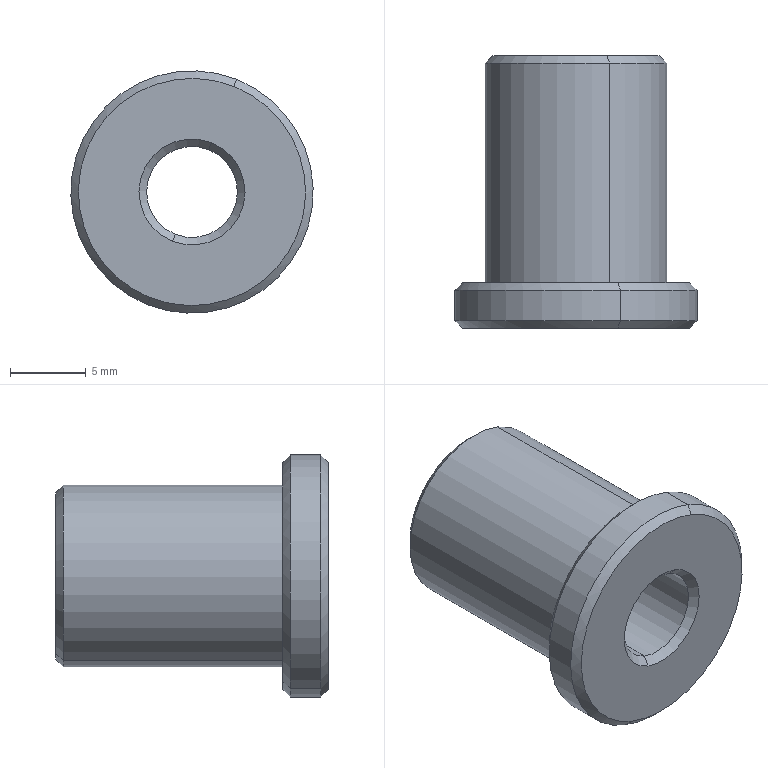Component | SolidWorks | GbgbSleeve-1 | 1 solid | 19 faces | box 16 x 18 x 16 mm | volume 1769 mm3 | cone 10 | cylinder 6 | plane 3 | commonest cylinder face diameters 6 x2 12 x2 16 x2
build123d program:
from build123d import *

# Parameters (mm, degrees)
SKETCH1_R           = 8
BOSS_EXTRUDE1_DEPTH = 3
SKETCH2_R           = 6
BOSS_EXTRUDE2_DEPTH = 15
SKETCH3_R           = 3
CUT_EXTRUDE1_DEPTH  = 22.26
CHAMFER1_SIZE       = 0.5


with BuildPart() as part:
    # Sketch1 → Boss-Extrude1 (new body)
    with BuildSketch(Plane(origin=(0, 0, 0), x_dir=(1, 0, 0), z_dir=(0, 1, 0))):
        with Locations(Location((0, 0, 0), (0, 0, 270))):
            Circle(SKETCH1_R)
    extrude(amount=BOSS_EXTRUDE1_DEPTH)

    # Sketch2 → Boss-Extrude2 (add)
    with BuildSketch(Plane(origin=(0, 3, 0), x_dir=(1, 0, 0), z_dir=(0, 1, 0))):
        with Locations(Location((0, 0, 0), (0, 0, 270))):
            Circle(SKETCH2_R)
    extrude(amount=BOSS_EXTRUDE2_DEPTH)

    # Sketch3 → Cut-Extrude1 (cut, through all)
    with BuildSketch(Plane(origin=(0, 18, 0), x_dir=(1, 0, 0), z_dir=(0, 1, 0))):
        with Locations(Location((0, 0, 0), (0, 0, 270))):
            Circle(SKETCH3_R)
    extrude(amount=-CUT_EXTRUDE1_DEPTH, mode=Mode.SUBTRACT)

    # Chamfer1
    chamfer1_edges = [part.edges().sort_by_distance(p)[0] for p in [
        (0, 0, -3),
        (0, 18, -3),
        (0, 0, -8),
        (0, 3, -8),
        (0, 18, -6),
    ]]
    chamfer(chamfer1_edges, length=CHAMFER1_SIZE)


solid = part.part

# Placed as in the assembly
solid = solid.moved(Location((55.446, 369.44, 430.232), (0, 0, 0)))
STEP:
#1=COLOUR_RGB('',0.7922,0.8196,0.9333);
#2=FILL_AREA_STYLE_COLOUR('',#1);
#3=FILL_AREA_STYLE('',(#2));
#4=SURFACE_STYLE_FILL_AREA(#3);
#5=SURFACE_SIDE_STYLE('',(#4));
#6=SURFACE_STYLE_USAGE(.BOTH.,#5);
#7=PRESENTATION_STYLE_ASSIGNMENT((#6));
#8=CARTESIAN_POINT('',(2.263,15.254,17.14));
#9=VERTEX_POINT('',#8);
#10=CARTESIAN_POINT('',(2.103,15.254,16.737));
#11=VERTEX_POINT('',#10);
#12=CARTESIAN_POINT('',(2.183,15.254,16.938));
#13=DIRECTION('',(-0.,1.,0.));
#14=DIRECTION('',(0.3675,0.,0.93));
#15=AXIS2_PLACEMENT_3D('',#12,#13,#14);
#16=CIRCLE('',#15,0.2165);
#17=EDGE_CURVE('',#9,#11,#16,.T.);
#18=ORIENTED_EDGE('',*,*,#17,.F.);
#19=CARTESIAN_POINT('',(2.27,15.234,17.158));
#20=VERTEX_POINT('',#19);
#21=CARTESIAN_POINT('',(2.263,15.254,17.14));
#22=DIRECTION('',(0.2599,-0.7071,0.6576));
#23=VECTOR('',#22,39.37);
#24=LINE('',#21,#23);
#25=EDGE_CURVE('',#9,#20,#24,.T.);
#26=ORIENTED_EDGE('',*,*,#25,.T.);
#27=CARTESIAN_POINT('',(2.096,15.234,16.719));
#28=VERTEX_POINT('',#27);
#29=CARTESIAN_POINT('',(2.183,15.234,16.938));
#30=DIRECTION('',(0.,-1.,-0.));
#31=DIRECTION('',(0.3675,0.,0.93));
#32=AXIS2_PLACEMENT_3D('',#29,#30,#31);
#33=CIRCLE('',#32,0.2362);
#34=EDGE_CURVE('',#28,#20,#33,.T.);
#35=ORIENTED_EDGE('',*,*,#34,.F.);
#36=CARTESIAN_POINT('',(2.103,15.254,16.737));
#37=DIRECTION('',(-0.2599,-0.7071,-0.6576));
#38=VECTOR('',#37,39.37);
#39=LINE('',#36,#38);
#40=EDGE_CURVE('',#11,#28,#39,.T.);
#41=ORIENTED_EDGE('',*,*,#40,.F.);
#42=EDGE_LOOP('',(#18,#26,#35,#41));
#43=FACE_OUTER_BOUND('',#42,.T.);
#44=CARTESIAN_POINT('',(2.183,15.254,16.938));
#45=DIRECTION('',(0.,-1.,-0.));
#46=DIRECTION('',(-0.3675,0.,-0.93));
#47=AXIS2_PLACEMENT_3D('',#44,#45,#46);
#48=CONICAL_SURFACE('',#47,0.2165,0.7854);
#49=ADVANCED_FACE('',(#43),#48,.T.);
#50=CARTESIAN_POINT('',(2.291,14.663,17.213));
#51=VERTEX_POINT('',#50);
#52=CARTESIAN_POINT('',(2.074,14.663,16.664));
#53=VERTEX_POINT('',#52);
#54=CARTESIAN_POINT('',(2.183,14.663,16.938));
#55=DIRECTION('',(-0.,1.,0.));
#56=DIRECTION('',(0.3675,0.,0.93));
#57=AXIS2_PLACEMENT_3D('',#54,#55,#56);
#58=CIRCLE('',#57,0.2953);
#59=EDGE_CURVE('',#51,#53,#58,.T.);
#60=ORIENTED_EDGE('',*,*,#59,.F.);
#61=CARTESIAN_POINT('',(2.299,14.643,17.231));
#62=VERTEX_POINT('',#61);
#63=CARTESIAN_POINT('',(2.291,14.663,17.213));
#64=DIRECTION('',(0.2599,-0.7071,0.6576));
#65=VECTOR('',#64,39.37);
#66=LINE('',#63,#65);
#67=EDGE_CURVE('',#51,#62,#66,.T.);
#68=ORIENTED_EDGE('',*,*,#67,.T.);
#69=CARTESIAN_POINT('',(2.067,14.643,16.645));
#70=VERTEX_POINT('',#69);
#71=CARTESIAN_POINT('',(2.183,14.643,16.938));
#72=DIRECTION('',(0.,-1.,-0.));
#73=DIRECTION('',(0.3675,0.,0.93));
#74=AXIS2_PLACEMENT_3D('',#71,#72,#73);
#75=CIRCLE('',#74,0.315);
#76=EDGE_CURVE('',#70,#62,#75,.T.);
#77=ORIENTED_EDGE('',*,*,#76,.F.);
#78=CARTESIAN_POINT('',(2.074,14.663,16.664));
#79=DIRECTION('',(-0.2599,-0.7071,-0.6576));
#80=VECTOR('',#79,39.37);
#81=LINE('',#78,#80);
#82=EDGE_CURVE('',#53,#70,#81,.T.);
#83=ORIENTED_EDGE('',*,*,#82,.F.);
#84=EDGE_LOOP('',(#60,#68,#77,#83));
#85=FACE_OUTER_BOUND('',#84,.T.);
#86=CARTESIAN_POINT('',(2.183,14.663,16.938));
#87=DIRECTION('',(0.,-1.,-0.));
#88=DIRECTION('',(-0.3675,0.,-0.93));
#89=AXIS2_PLACEMENT_3D('',#86,#87,#88);
#90=CONICAL_SURFACE('',#89,0.2953,0.7854);
#91=ADVANCED_FACE('',(#85),#90,.T.);
#92=CARTESIAN_POINT('',(2.074,14.545,16.664));
#93=VERTEX_POINT('',#92);
#94=CARTESIAN_POINT('',(2.291,14.545,17.213));
#95=VERTEX_POINT('',#94);
#96=CARTESIAN_POINT('',(2.183,14.545,16.938));
#97=DIRECTION('',(0.,-1.,-0.));
#98=DIRECTION('',(0.3675,0.,0.93));
#99=AXIS2_PLACEMENT_3D('',#96,#97,#98);
#100=CIRCLE('',#99,0.2953);
#101=EDGE_CURVE('',#93,#95,#100,.T.);
#102=ORIENTED_EDGE('',*,*,#101,.F.);
#103=CARTESIAN_POINT('',(2.067,14.565,16.645));
#104=VERTEX_POINT('',#103);
#105=CARTESIAN_POINT('',(2.067,14.565,16.645));
#106=DIRECTION('',(-0.2599,0.7071,-0.6576));
#107=VECTOR('',#106,39.37);
#108=LINE('',#105,#107);
#109=EDGE_CURVE('',#93,#104,#108,.T.);
#110=ORIENTED_EDGE('',*,*,#109,.T.);
#111=CARTESIAN_POINT('',(2.299,14.565,17.231));
#112=VERTEX_POINT('',#111);
#113=CARTESIAN_POINT('',(2.183,14.565,16.938));
#114=DIRECTION('',(-0.,1.,0.));
#115=DIRECTION('',(0.3675,0.,0.93));
#116=AXIS2_PLACEMENT_3D('',#113,#114,#115);
#117=CIRCLE('',#116,0.315);
#118=EDGE_CURVE('',#112,#104,#117,.T.);
#119=ORIENTED_EDGE('',*,*,#118,.F.);
#120=CARTESIAN_POINT('',(2.299,14.565,17.231));
#121=DIRECTION('',(0.2599,0.7071,0.6576));
#122=VECTOR('',#121,39.37);
#123=LINE('',#120,#122);
#124=EDGE_CURVE('',#95,#112,#123,.T.);
#125=ORIENTED_EDGE('',*,*,#124,.F.);
#126=EDGE_LOOP('',(#102,#110,#119,#125));
#127=FACE_OUTER_BOUND('',#126,.T.);
#128=CARTESIAN_POINT('',(2.183,14.565,16.938));
#129=DIRECTION('',(-0.,1.,0.));
#130=DIRECTION('',(0.3675,0.,0.93));
#131=AXIS2_PLACEMENT_3D('',#128,#129,#130);
#132=CONICAL_SURFACE('',#131,0.315,0.7854);
#133=ADVANCED_FACE('',(#127),#132,.T.);
#134=CARTESIAN_POINT('',(2.226,14.565,17.048));
#135=VERTEX_POINT('',#134);
#136=CARTESIAN_POINT('',(2.14,14.565,16.828));
#137=VERTEX_POINT('',#136);
#138=CARTESIAN_POINT('',(2.183,14.565,16.938));
#139=DIRECTION('',(0.,-1.,-0.));
#140=DIRECTION('',(0.3675,0.,0.93));
#141=AXIS2_PLACEMENT_3D('',#138,#139,#140);
#142=CIRCLE('',#141,0.1181);
#143=EDGE_CURVE('',#135,#137,#142,.T.);
#144=ORIENTED_EDGE('',*,*,#143,.F.);
#145=CARTESIAN_POINT('',(2.234,14.545,17.066));
#146=VERTEX_POINT('',#145);
#147=CARTESIAN_POINT('',(2.234,14.545,17.066));
#148=DIRECTION('',(0.2599,-0.7071,0.6576));
#149=VECTOR('',#148,39.37);
#150=LINE('',#147,#149);
#151=EDGE_CURVE('',#135,#146,#150,.T.);
#152=ORIENTED_EDGE('',*,*,#151,.T.);
#153=CARTESIAN_POINT('',(2.132,14.545,16.81));
#154=VERTEX_POINT('',#153);
#155=CARTESIAN_POINT('',(2.183,14.545,16.938));
#156=DIRECTION('',(-0.,1.,0.));
#157=DIRECTION('',(0.3675,0.,0.93));
#158=AXIS2_PLACEMENT_3D('',#155,#156,#157);
#159=CIRCLE('',#158,0.1378);
#160=EDGE_CURVE('',#154,#146,#159,.T.);
#161=ORIENTED_EDGE('',*,*,#160,.F.);
#162=CARTESIAN_POINT('',(2.132,14.545,16.81));
#163=DIRECTION('',(-0.2599,-0.7071,-0.6576));
#164=VECTOR('',#163,39.37);
#165=LINE('',#162,#164);
#166=EDGE_CURVE('',#137,#154,#165,.T.);
#167=ORIENTED_EDGE('',*,*,#166,.F.);
#168=EDGE_LOOP('',(#144,#152,#161,#167));
#169=FACE_OUTER_BOUND('',#168,.T.);
#170=CARTESIAN_POINT('',(2.183,14.545,16.938));
#171=DIRECTION('',(0.,-1.,-0.));
#172=DIRECTION('',(-0.3675,0.,-0.93));
#173=AXIS2_PLACEMENT_3D('',#170,#171,#172);
#174=CONICAL_SURFACE('',#173,0.1378,0.7854);
#175=ADVANCED_FACE('',(#169),#174,.F.);
#176=CARTESIAN_POINT('',(2.14,15.234,16.828));
#177=VERTEX_POINT('',#176);
#178=CARTESIAN_POINT('',(2.226,15.234,17.048));
#179=VERTEX_POINT('',#178);
#180=CARTESIAN_POINT('',(2.183,15.234,16.938));
#181=DIRECTION('',(-0.,1.,0.));
#182=DIRECTION('',(0.3675,0.,0.93));
#183=AXIS2_PLACEMENT_3D('',#180,#181,#182);
#184=CIRCLE('',#183,0.1181);
#185=EDGE_CURVE('',#177,#179,#184,.T.);
#186=ORIENTED_EDGE('',*,*,#185,.F.);
#187=CARTESIAN_POINT('',(2.132,15.254,16.81));
#188=VERTEX_POINT('',#187);
#189=CARTESIAN_POINT('',(2.14,15.234,16.828));
#190=DIRECTION('',(-0.2599,0.7071,-0.6576));
#191=VECTOR('',#190,39.37);
#192=LINE('',#189,#191);
#193=EDGE_CURVE('',#177,#188,#192,.T.);
#194=ORIENTED_EDGE('',*,*,#193,.T.);
#195=CARTESIAN_POINT('',(2.234,15.254,17.066));
#196=VERTEX_POINT('',#195);
#197=CARTESIAN_POINT('',(2.183,15.254,16.938));
#198=DIRECTION('',(0.,-1.,-0.));
#199=DIRECTION('',(0.3675,0.,0.93));
#200=AXIS2_PLACEMENT_3D('',#197,#198,#199);
#201=CIRCLE('',#200,0.1378);
#202=EDGE_CURVE('',#196,#188,#201,.T.);
#203=ORIENTED_EDGE('',*,*,#202,.F.);
#204=CARTESIAN_POINT('',(2.226,15.234,17.048));
#205=DIRECTION('',(0.2599,0.7071,0.6576));
#206=VECTOR('',#205,39.37);
#207=LINE('',#204,#206);
#208=EDGE_CURVE('',#179,#196,#207,.T.);
#209=ORIENTED_EDGE('',*,*,#208,.F.);
#210=EDGE_LOOP('',(#186,#194,#203,#209));
#211=FACE_OUTER_BOUND('',#210,.T.);
#212=CARTESIAN_POINT('',(2.183,15.234,16.938));
#213=DIRECTION('',(-0.,1.,0.));
#214=DIRECTION('',(0.3675,0.,0.93));
#215=AXIS2_PLACEMENT_3D('',#212,#213,#214);
#216=CONICAL_SURFACE('',#215,0.1181,0.7854);
#217=ADVANCED_FACE('',(#211),#216,.F.);
#218=ORIENTED_EDGE('',*,*,#143,.T.);
#219=CARTESIAN_POINT('',(2.14,14.545,16.828));
#220=DIRECTION('',(-0.,1.,0.));
#221=VECTOR('',#220,39.37);
#222=LINE('',#219,#221);
#223=EDGE_CURVE('',#137,#177,#222,.T.);
#224=ORIENTED_EDGE('',*,*,#223,.T.);
#225=ORIENTED_EDGE('',*,*,#185,.T.);
#226=CARTESIAN_POINT('',(2.226,14.545,17.048));
#227=DIRECTION('',(-0.,1.,0.));
#228=VECTOR('',#227,39.37);
#229=LINE('',#226,#228);
#230=EDGE_CURVE('',#135,#179,#229,.T.);
#231=ORIENTED_EDGE('',*,*,#230,.F.);
#232=EDGE_LOOP('',(#218,#224,#225,#231));
#233=FACE_OUTER_BOUND('',#232,.T.);
#234=CARTESIAN_POINT('',(2.183,14.545,16.938));
#235=DIRECTION('',(-0.,1.,0.));
#236=DIRECTION('',(0.3675,0.,0.93));
#237=AXIS2_PLACEMENT_3D('',#234,#235,#236);
#238=CYLINDRICAL_SURFACE('',#237,0.1181);
#239=ADVANCED_FACE('',(#233),#238,.F.);
#240=ORIENTED_EDGE('',*,*,#34,.T.);
#241=CARTESIAN_POINT('',(2.27,14.663,17.158));
#242=VERTEX_POINT('',#241);
#243=CARTESIAN_POINT('',(2.27,15.254,17.158));
#244=DIRECTION('',(0.,-1.,-0.));
#245=VECTOR('',#244,39.37);
#246=LINE('',#243,#245);
#247=EDGE_CURVE('',#20,#242,#246,.T.);
#248=ORIENTED_EDGE('',*,*,#247,.T.);
#249=CARTESIAN_POINT('',(2.096,14.663,16.719));
#250=VERTEX_POINT('',#249);
#251=CARTESIAN_POINT('',(2.183,14.663,16.938));
#252=DIRECTION('',(-0.,1.,0.));
#253=DIRECTION('',(0.3675,0.,0.93));
#254=AXIS2_PLACEMENT_3D('',#251,#252,#253);
#255=CIRCLE('',#254,0.2362);
#256=EDGE_CURVE('',#242,#250,#255,.T.);
#257=ORIENTED_EDGE('',*,*,#256,.T.);
#258=CARTESIAN_POINT('',(2.096,15.254,16.719));
#259=DIRECTION('',(0.,-1.,-0.));
#260=VECTOR('',#259,39.37);
#261=LINE('',#258,#260);
#262=EDGE_CURVE('',#28,#250,#261,.T.);
#263=ORIENTED_EDGE('',*,*,#262,.F.);
#264=EDGE_LOOP('',(#240,#248,#257,#263));
#265=FACE_OUTER_BOUND('',#264,.T.);
#266=CARTESIAN_POINT('',(2.183,15.254,16.938));
#267=DIRECTION('',(0.,-1.,-0.));
#268=DIRECTION('',(-0.3675,0.,-0.93));
#269=AXIS2_PLACEMENT_3D('',#266,#267,#268);
#270=CYLINDRICAL_SURFACE('',#269,0.2362);
#271=ADVANCED_FACE('',(#265),#270,.T.);
#272=ORIENTED_EDGE('',*,*,#76,.T.);
#273=CARTESIAN_POINT('',(2.299,14.663,17.231));
#274=DIRECTION('',(0.,-1.,-0.));
#275=VECTOR('',#274,39.37);
#276=LINE('',#273,#275);
#277=EDGE_CURVE('',#62,#112,#276,.T.);
#278=ORIENTED_EDGE('',*,*,#277,.T.);
#279=ORIENTED_EDGE('',*,*,#118,.T.);
#280=CARTESIAN_POINT('',(2.067,14.663,16.645));
#281=DIRECTION('',(0.,-1.,-0.));
#282=VECTOR('',#281,39.37);
#283=LINE('',#280,#282);
#284=EDGE_CURVE('',#70,#104,#283,.T.);
#285=ORIENTED_EDGE('',*,*,#284,.F.);
#286=EDGE_LOOP('',(#272,#278,#279,#285));
#287=FACE_OUTER_BOUND('',#286,.T.);
#288=CARTESIAN_POINT('',(2.183,14.663,16.938));
#289=DIRECTION('',(0.,-1.,-0.));
#290=DIRECTION('',(-0.3675,0.,-0.93));
#291=AXIS2_PLACEMENT_3D('',#288,#289,#290);
#292=CYLINDRICAL_SURFACE('',#291,0.315);
#293=ADVANCED_FACE('',(#287),#292,.T.);
#294=CARTESIAN_POINT('',(2.183,14.663,16.938));
#295=DIRECTION('',(-0.,1.,0.));
#296=DIRECTION('',(0.3675,0.,0.93));
#297=AXIS2_PLACEMENT_3D('',#294,#295,#296);
#298=CIRCLE('',#297,0.2953);
#299=EDGE_CURVE('',#53,#51,#298,.T.);
#300=ORIENTED_EDGE('',*,*,#299,.T.);
#301=ORIENTED_EDGE('',*,*,#59,.T.);
#302=EDGE_LOOP('',(#300,#301));
#303=FACE_OUTER_BOUND('',#302,.T.);
#304=CARTESIAN_POINT('',(2.183,14.663,16.938));
#305=DIRECTION('',(-0.,1.,0.));
#306=DIRECTION('',(0.3675,0.,0.93));
#307=AXIS2_PLACEMENT_3D('',#304,#305,#306);
#308=CIRCLE('',#307,0.2362);
#309=EDGE_CURVE('',#250,#242,#308,.T.);
#310=ORIENTED_EDGE('',*,*,#309,.F.);
#311=ORIENTED_EDGE('',*,*,#256,.F.);
#312=EDGE_LOOP('',(#310,#311));
#313=FACE_BOUND('',#312,.T.);
#314=CARTESIAN_POINT('',(2.183,14.663,16.938));
#315=DIRECTION('',(-0.,1.,0.));
#316=DIRECTION('',(0.3675,-0.,0.93));
#317=AXIS2_PLACEMENT_3D('',#314,#315,#316);
#318=PLANE('',#317);
#319=ADVANCED_FACE('',(#303,#313),#318,.T.);
#320=ORIENTED_EDGE('',*,*,#277,.F.);
#321=CARTESIAN_POINT('',(2.183,14.643,16.938));
#322=DIRECTION('',(0.,-1.,-0.));
#323=DIRECTION('',(0.3675,0.,0.93));
#324=AXIS2_PLACEMENT_3D('',#321,#322,#323);
#325=CIRCLE('',#324,0.315);
#326=EDGE_CURVE('',#62,#70,#325,.T.);
#327=ORIENTED_EDGE('',*,*,#326,.T.);
#328=ORIENTED_EDGE('',*,*,#284,.T.);
#329=CARTESIAN_POINT('',(2.183,14.565,16.938));
#330=DIRECTION('',(-0.,1.,0.));
#331=DIRECTION('',(0.3675,0.,0.93));
#332=AXIS2_PLACEMENT_3D('',#329,#330,#331);
#333=CIRCLE('',#332,0.315);
#334=EDGE_CURVE('',#104,#112,#333,.T.);
#335=ORIENTED_EDGE('',*,*,#334,.T.);
#336=EDGE_LOOP('',(#320,#327,#328,#335));
#337=FACE_OUTER_BOUND('',#336,.T.);
#338=CARTESIAN_POINT('',(2.183,14.663,16.938));
#339=DIRECTION('',(0.,-1.,-0.));
#340=DIRECTION('',(-0.3675,0.,-0.93));
#341=AXIS2_PLACEMENT_3D('',#338,#339,#340);
#342=CYLINDRICAL_SURFACE('',#341,0.315);
#343=ADVANCED_FACE('',(#337),#342,.T.);
#344=ORIENTED_EDGE('',*,*,#160,.T.);
#345=CARTESIAN_POINT('',(2.183,14.545,16.938));
#346=DIRECTION('',(-0.,1.,0.));
#347=DIRECTION('',(0.3675,0.,0.93));
#348=AXIS2_PLACEMENT_3D('',#345,#346,#347);
#349=CIRCLE('',#348,0.1378);
#350=EDGE_CURVE('',#146,#154,#349,.T.);
#351=ORIENTED_EDGE('',*,*,#350,.T.);
#352=EDGE_LOOP('',(#344,#351));
#353=FACE_BOUND('',#352,.T.);
#354=CARTESIAN_POINT('',(2.183,14.545,16.938));
#355=DIRECTION('',(0.,-1.,-0.));
#356=DIRECTION('',(0.3675,0.,0.93));
#357=AXIS2_PLACEMENT_3D('',#354,#355,#356);
#358=CIRCLE('',#357,0.2953);
#359=EDGE_CURVE('',#95,#93,#358,.T.);
#360=ORIENTED_EDGE('',*,*,#359,.T.);
#361=ORIENTED_EDGE('',*,*,#101,.T.);
#362=EDGE_LOOP('',(#360,#361));
#363=FACE_OUTER_BOUND('',#362,.T.);
#364=CARTESIAN_POINT('',(2.183,14.545,16.938));
#365=DIRECTION('',(-0.,1.,0.));
#366=DIRECTION('',(0.3675,-0.,0.93));
#367=AXIS2_PLACEMENT_3D('',#364,#365,#366);
#368=PLANE('',#367);
#369=ADVANCED_FACE('',(#353,#363),#368,.F.);
#370=ORIENTED_EDGE('',*,*,#247,.F.);
#371=CARTESIAN_POINT('',(2.183,15.234,16.938));
#372=DIRECTION('',(0.,-1.,-0.));
#373=DIRECTION('',(0.3675,0.,0.93));
#374=AXIS2_PLACEMENT_3D('',#371,#372,#373);
#375=CIRCLE('',#374,0.2362);
#376=EDGE_CURVE('',#20,#28,#375,.T.);
#377=ORIENTED_EDGE('',*,*,#376,.T.);
#378=ORIENTED_EDGE('',*,*,#262,.T.);
#379=ORIENTED_EDGE('',*,*,#309,.T.);
#380=EDGE_LOOP('',(#370,#377,#378,#379));
#381=FACE_OUTER_BOUND('',#380,.T.);
#382=CARTESIAN_POINT('',(2.183,15.254,16.938));
#383=DIRECTION('',(0.,-1.,-0.));
#384=DIRECTION('',(-0.3675,0.,-0.93));
#385=AXIS2_PLACEMENT_3D('',#382,#383,#384);
#386=CYLINDRICAL_SURFACE('',#385,0.2362);
#387=ADVANCED_FACE('',(#381),#386,.T.);
#388=ORIENTED_EDGE('',*,*,#202,.T.);
#389=CARTESIAN_POINT('',(2.183,15.254,16.938));
#390=DIRECTION('',(0.,-1.,-0.));
#391=DIRECTION('',(0.3675,0.,0.93));
#392=AXIS2_PLACEMENT_3D('',#389,#390,#391);
#393=CIRCLE('',#392,0.1378);
#394=EDGE_CURVE('',#188,#196,#393,.T.);
#395=ORIENTED_EDGE('',*,*,#394,.T.);
#396=EDGE_LOOP('',(#388,#395));
#397=FACE_BOUND('',#396,.T.);
#398=CARTESIAN_POINT('',(2.183,15.254,16.938));
#399=DIRECTION('',(-0.,1.,0.));
#400=DIRECTION('',(0.3675,0.,0.93));
#401=AXIS2_PLACEMENT_3D('',#398,#399,#400);
#402=CIRCLE('',#401,0.2165);
#403=EDGE_CURVE('',#11,#9,#402,.T.);
#404=ORIENTED_EDGE('',*,*,#403,.T.);
#405=ORIENTED_EDGE('',*,*,#17,.T.);
#406=EDGE_LOOP('',(#404,#405));
#407=FACE_OUTER_BOUND('',#406,.T.);
#408=CARTESIAN_POINT('',(2.183,15.254,16.938));
#409=DIRECTION('',(-0.,1.,0.));
#410=DIRECTION('',(0.3675,-0.,0.93));
#411=AXIS2_PLACEMENT_3D('',#408,#409,#410);
#412=PLANE('',#411);
#413=ADVANCED_FACE('',(#397,#407),#412,.T.);
#414=ORIENTED_EDGE('',*,*,#223,.F.);
#415=CARTESIAN_POINT('',(2.183,14.565,16.938));
#416=DIRECTION('',(0.,-1.,-0.));
#417=DIRECTION('',(0.3675,0.,0.93));
#418=AXIS2_PLACEMENT_3D('',#415,#416,#417);
#419=CIRCLE('',#418,0.1181);
#420=EDGE_CURVE('',#137,#135,#419,.T.);
#421=ORIENTED_EDGE('',*,*,#420,.T.);
#422=ORIENTED_EDGE('',*,*,#230,.T.);
#423=CARTESIAN_POINT('',(2.183,15.234,16.938));
#424=DIRECTION('',(-0.,1.,0.));
#425=DIRECTION('',(0.3675,0.,0.93));
#426=AXIS2_PLACEMENT_3D('',#423,#424,#425);
#427=CIRCLE('',#426,0.1181);
#428=EDGE_CURVE('',#179,#177,#427,.T.);
#429=ORIENTED_EDGE('',*,*,#428,.T.);
#430=EDGE_LOOP('',(#414,#421,#422,#429));
#431=FACE_OUTER_BOUND('',#430,.T.);
#432=CARTESIAN_POINT('',(2.183,14.545,16.938));
#433=DIRECTION('',(-0.,1.,0.));
#434=DIRECTION('',(0.3675,0.,0.93));
#435=AXIS2_PLACEMENT_3D('',#432,#433,#434);
#436=CYLINDRICAL_SURFACE('',#435,0.1181);
#437=ADVANCED_FACE('',(#431),#436,.F.);
#438=ORIENTED_EDGE('',*,*,#193,.F.);
#439=ORIENTED_EDGE('',*,*,#428,.F.);
#440=ORIENTED_EDGE('',*,*,#208,.T.);
#441=ORIENTED_EDGE('',*,*,#394,.F.);
#442=EDGE_LOOP('',(#438,#439,#440,#441));
#443=FACE_OUTER_BOUND('',#442,.T.);
#444=CARTESIAN_POINT('',(2.183,15.234,16.938));
#445=DIRECTION('',(-0.,1.,0.));
#446=DIRECTION('',(0.3675,0.,0.93));
#447=AXIS2_PLACEMENT_3D('',#444,#445,#446);
#448=CONICAL_SURFACE('',#447,0.1181,0.7854);
#449=ADVANCED_FACE('',(#443),#448,.F.);
#450=ORIENTED_EDGE('',*,*,#151,.F.);
#451=ORIENTED_EDGE('',*,*,#420,.F.);
#452=ORIENTED_EDGE('',*,*,#166,.T.);
#453=ORIENTED_EDGE('',*,*,#350,.F.);
#454=EDGE_LOOP('',(#450,#451,#452,#453));
#455=FACE_OUTER_BOUND('',#454,.T.);
#456=CARTESIAN_POINT('',(2.183,14.545,16.938));
#457=DIRECTION('',(0.,-1.,-0.));
#458=DIRECTION('',(-0.3675,0.,-0.93));
#459=AXIS2_PLACEMENT_3D('',#456,#457,#458);
#460=CONICAL_SURFACE('',#459,0.1378,0.7854);
#461=ADVANCED_FACE('',(#455),#460,.F.);
#462=ORIENTED_EDGE('',*,*,#109,.F.);
#463=ORIENTED_EDGE('',*,*,#359,.F.);
#464=ORIENTED_EDGE('',*,*,#124,.T.);
#465=ORIENTED_EDGE('',*,*,#334,.F.);
#466=EDGE_LOOP('',(#462,#463,#464,#465));
#467=FACE_OUTER_BOUND('',#466,.T.);
#468=CARTESIAN_POINT('',(2.183,14.565,16.938));
#469=DIRECTION('',(-0.,1.,0.));
#470=DIRECTION('',(0.3675,0.,0.93));
#471=AXIS2_PLACEMENT_3D('',#468,#469,#470);
#472=CONICAL_SURFACE('',#471,0.315,0.7854);
#473=ADVANCED_FACE('',(#467),#472,.T.);
#474=ORIENTED_EDGE('',*,*,#67,.F.);
#475=ORIENTED_EDGE('',*,*,#299,.F.);
#476=ORIENTED_EDGE('',*,*,#82,.T.);
#477=ORIENTED_EDGE('',*,*,#326,.F.);
#478=EDGE_LOOP('',(#474,#475,#476,#477));
#479=FACE_OUTER_BOUND('',#478,.T.);
#480=CARTESIAN_POINT('',(2.183,14.663,16.938));
#481=DIRECTION('',(0.,-1.,-0.));
#482=DIRECTION('',(-0.3675,0.,-0.93));
#483=AXIS2_PLACEMENT_3D('',#480,#481,#482);
#484=CONICAL_SURFACE('',#483,0.2953,0.7854);
#485=ADVANCED_FACE('',(#479),#484,.T.);
#486=ORIENTED_EDGE('',*,*,#25,.F.);
#487=ORIENTED_EDGE('',*,*,#403,.F.);
#488=ORIENTED_EDGE('',*,*,#40,.T.);
#489=ORIENTED_EDGE('',*,*,#376,.F.);
#490=EDGE_LOOP('',(#486,#487,#488,#489));
#491=FACE_OUTER_BOUND('',#490,.T.);
#492=CARTESIAN_POINT('',(2.183,15.254,16.938));
#493=DIRECTION('',(0.,-1.,-0.));
#494=DIRECTION('',(-0.3675,0.,-0.93));
#495=AXIS2_PLACEMENT_3D('',#492,#493,#494);
#496=CONICAL_SURFACE('',#495,0.2165,0.7854);
#497=ADVANCED_FACE('',(#491),#496,.T.);
#498=CLOSED_SHELL('',(#49,#91,#133,#175,#217,#239,#271,#293,#319,#343,#369,#387,#413,#437,#449,#461,#473,#485,#497));
#499=MANIFOLD_SOLID_BREP('',#498);
#500=STYLED_ITEM('',(#7),#499);
#501=PRESENTATION_LAYER_ASSIGNMENT('','',(#500));
#502=(LENGTH_UNIT()NAMED_UNIT(*)SI_UNIT($,.METRE.));
#503=LENGTH_MEASURE_WITH_UNIT(LENGTH_MEASURE(0.0254),#502);
#504=DIMENSIONAL_EXPONENTS(1.,0.,0.,0.,0.,0.,0.);
#505=(CONVERSION_BASED_UNIT('',#503)LENGTH_UNIT()NAMED_UNIT(#504));
#506=UNCERTAINTY_MEASURE_WITH_UNIT(LENGTH_MEASURE(0.00001),#505,'','');
#507=(NAMED_UNIT(*)PLANE_ANGLE_UNIT()SI_UNIT($,.RADIAN.));
#508=(NAMED_UNIT(*)SI_UNIT($,.STERADIAN.)SOLID_ANGLE_UNIT());
#509=(GEOMETRIC_REPRESENTATION_CONTEXT(3)GLOBAL_UNCERTAINTY_ASSIGNED_CONTEXT((#506))GLOBAL_UNIT_ASSIGNED_CONTEXT((#505,#507,#508))REPRESENTATION_CONTEXT('',''));
#510=MECHANICAL_DESIGN_GEOMETRIC_PRESENTATION_REPRESENTATION('',(#500),#509);
#511=CARTESIAN_POINT('',(0.,0.,0.));
#512=DIRECTION('',(0.,0.,1.));
#513=DIRECTION('',(1.,0.,0.));
#514=AXIS2_PLACEMENT_3D('',#511,#512,#513);
#515=(LENGTH_UNIT()NAMED_UNIT(*)SI_UNIT($,.METRE.));
#516=LENGTH_MEASURE_WITH_UNIT(LENGTH_MEASURE(0.0254),#515);
#517=DIMENSIONAL_EXPONENTS(1.,0.,0.,0.,0.,0.,0.);
#518=(CONVERSION_BASED_UNIT('',#516)LENGTH_UNIT()NAMED_UNIT(#517));
#519=UNCERTAINTY_MEASURE_WITH_UNIT(LENGTH_MEASURE(0.00001),#518,'','');
#520=(NAMED_UNIT(*)PLANE_ANGLE_UNIT()SI_UNIT($,.RADIAN.));
#521=(NAMED_UNIT(*)SI_UNIT($,.STERADIAN.)SOLID_ANGLE_UNIT());
#522=(GEOMETRIC_REPRESENTATION_CONTEXT(3)GLOBAL_UNCERTAINTY_ASSIGNED_CONTEXT((#519))GLOBAL_UNIT_ASSIGNED_CONTEXT((#518,#520,#521))REPRESENTATION_CONTEXT('',''));
#523=ADVANCED_BREP_SHAPE_REPRESENTATION('',(#499,#514),#522);